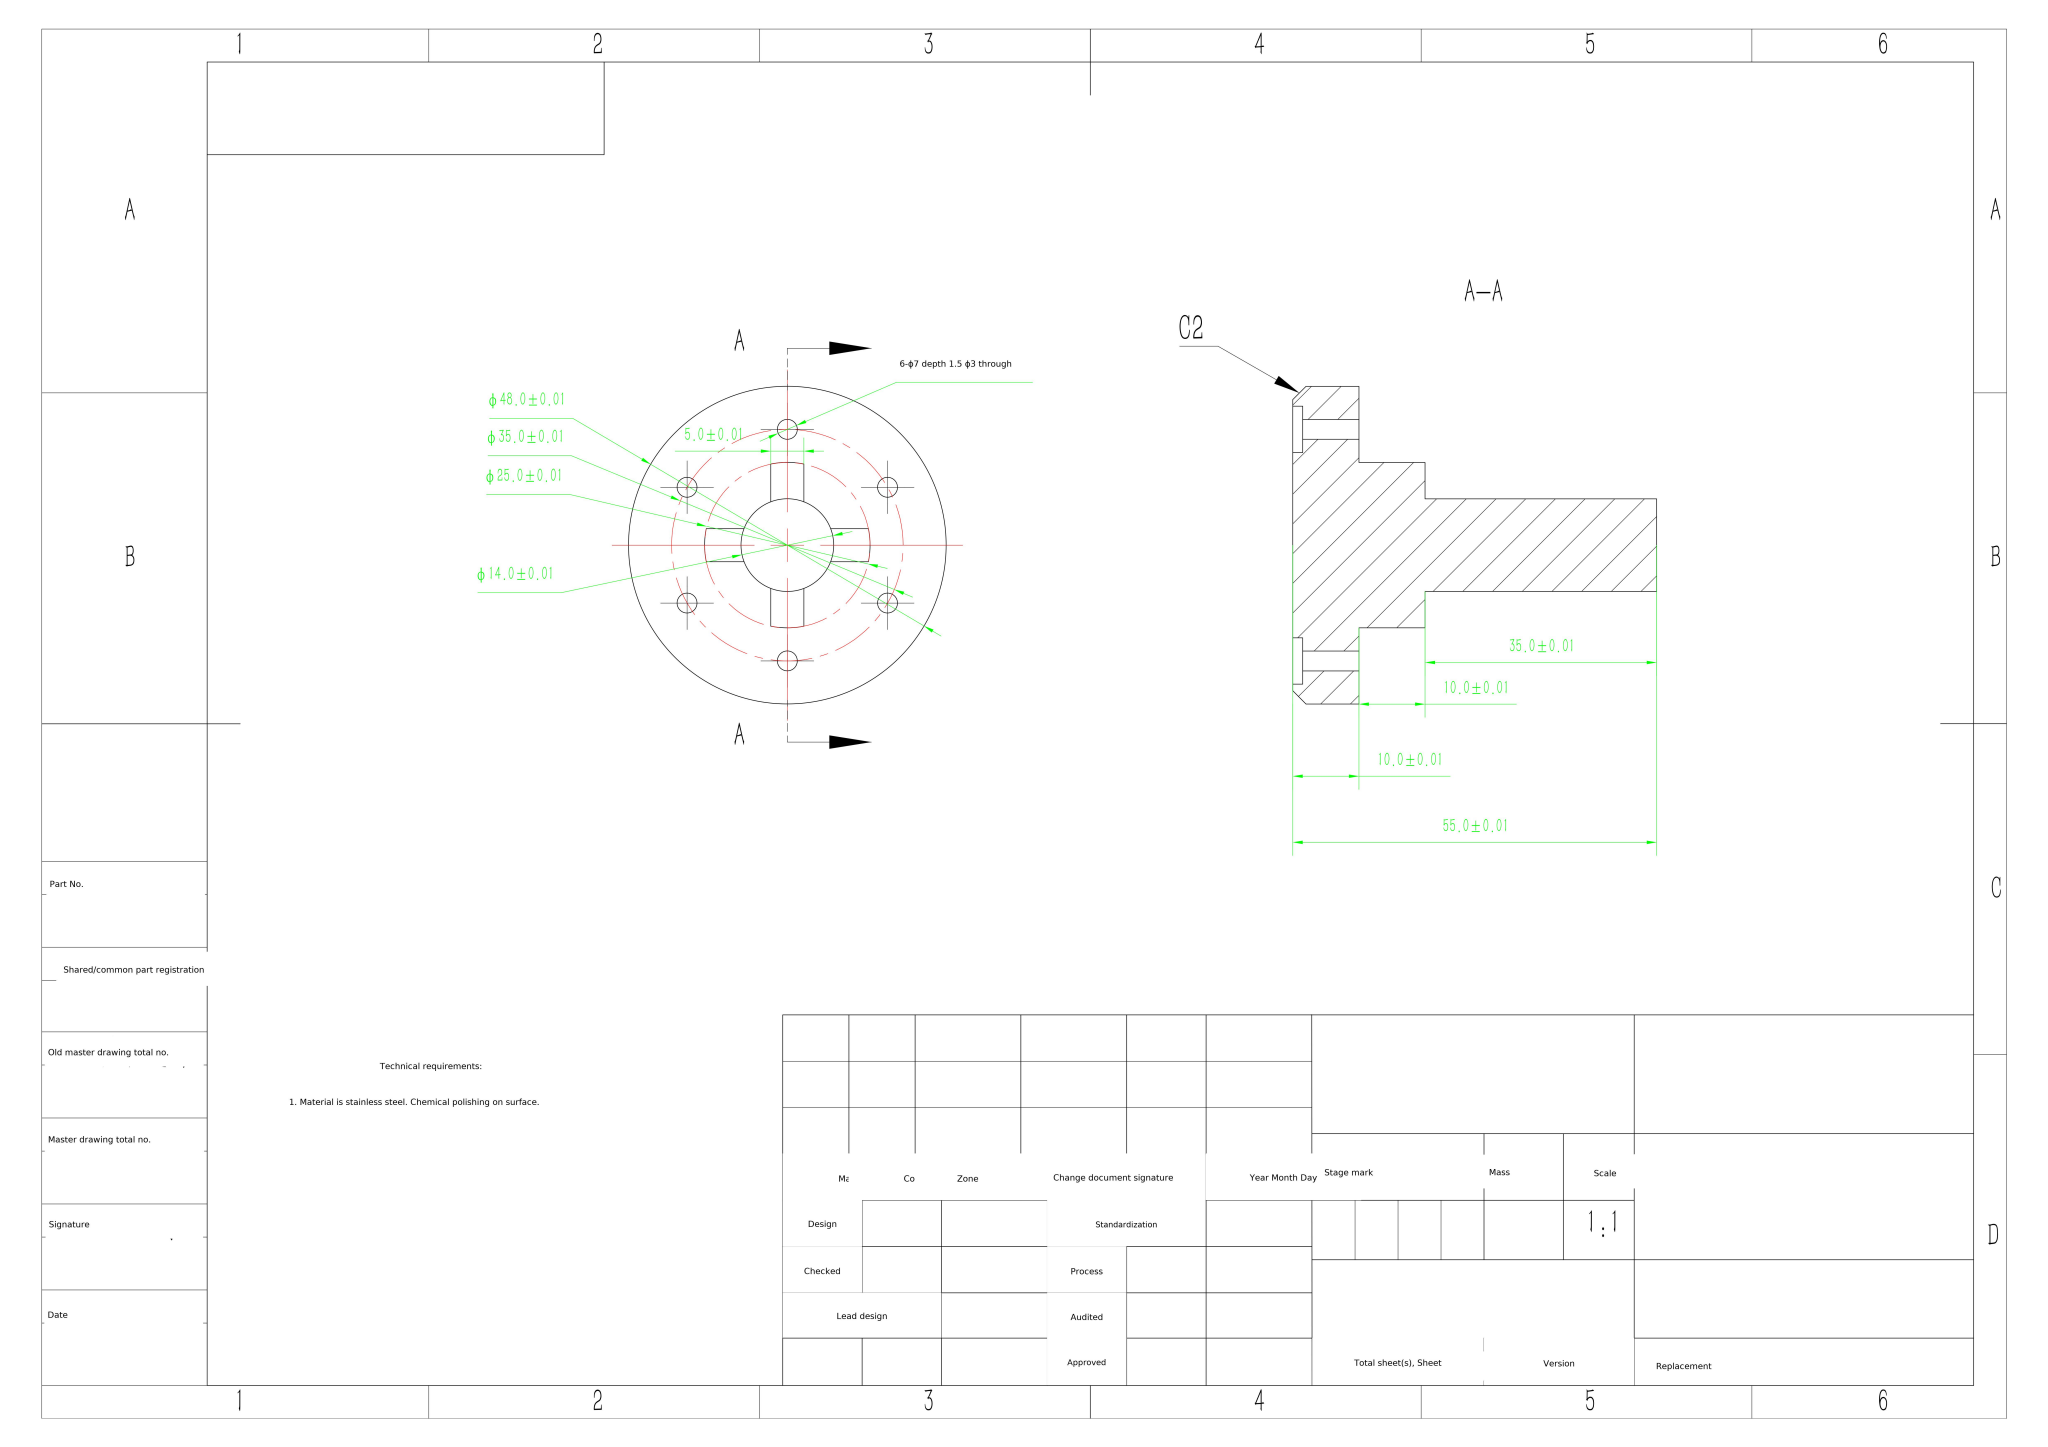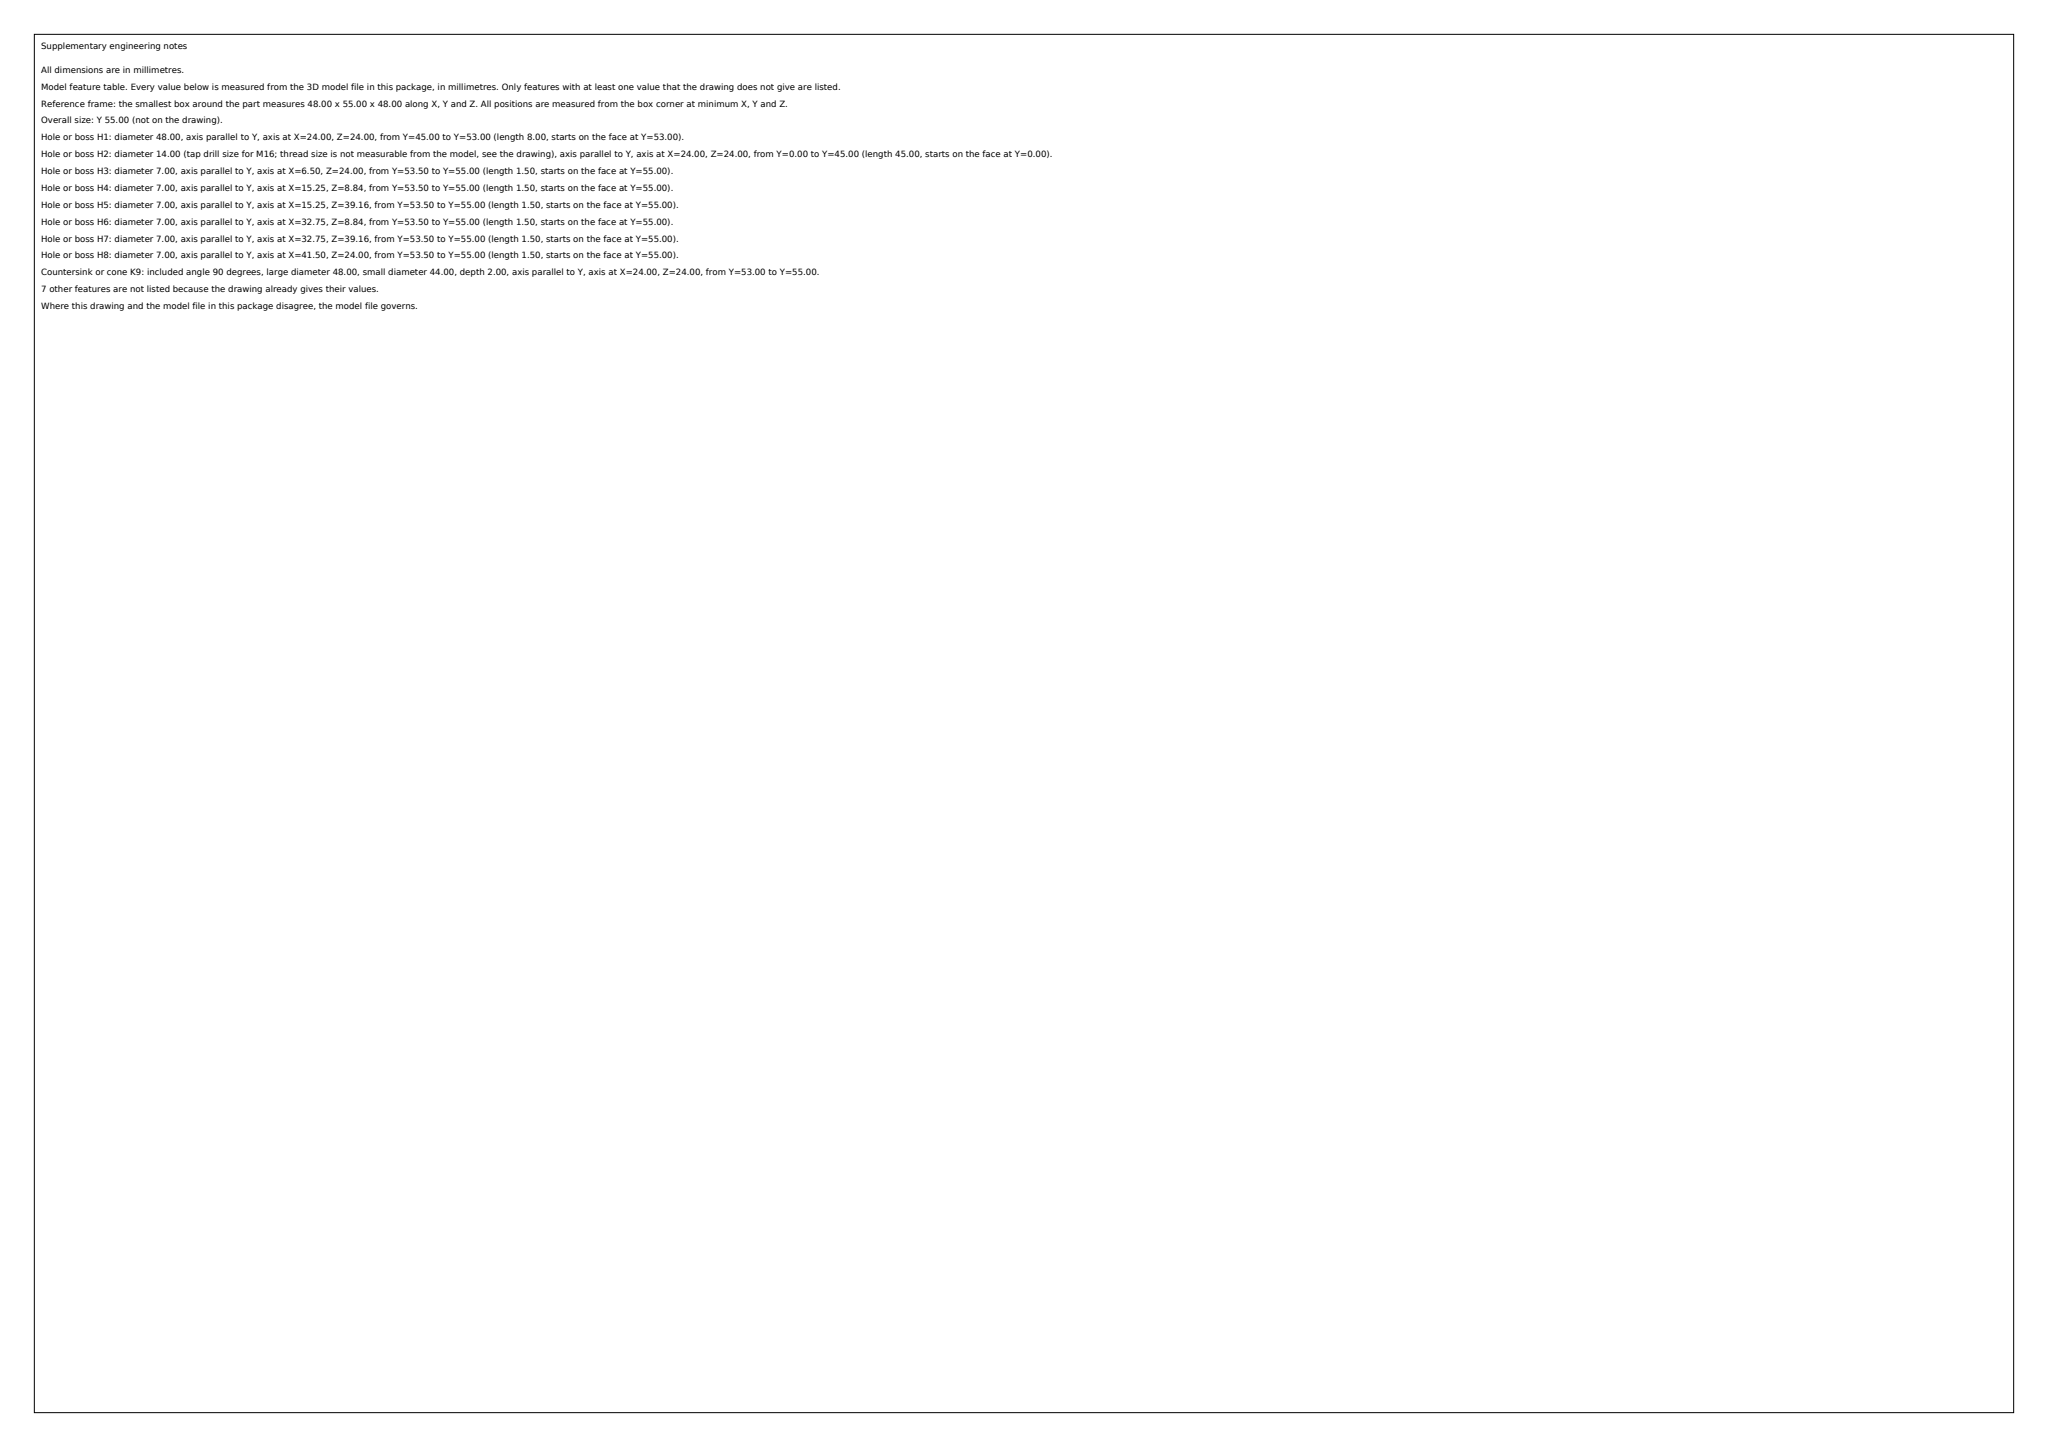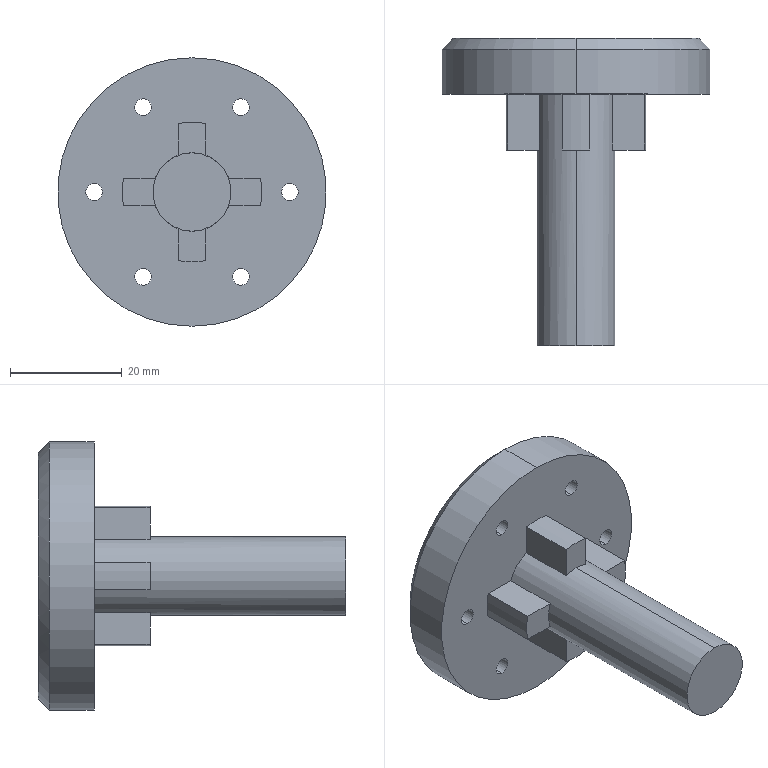Part | SolidWorks | mm | material stainless steel | 1 solid | 56 faces | box 48 x 55 x 48 mm | volume 25136 mm3 | cylinder 33 | plane 21 | cone 2 | commonest cylinder face diameters 3 x12 7 x12 25 x5 14 x2 48 x2